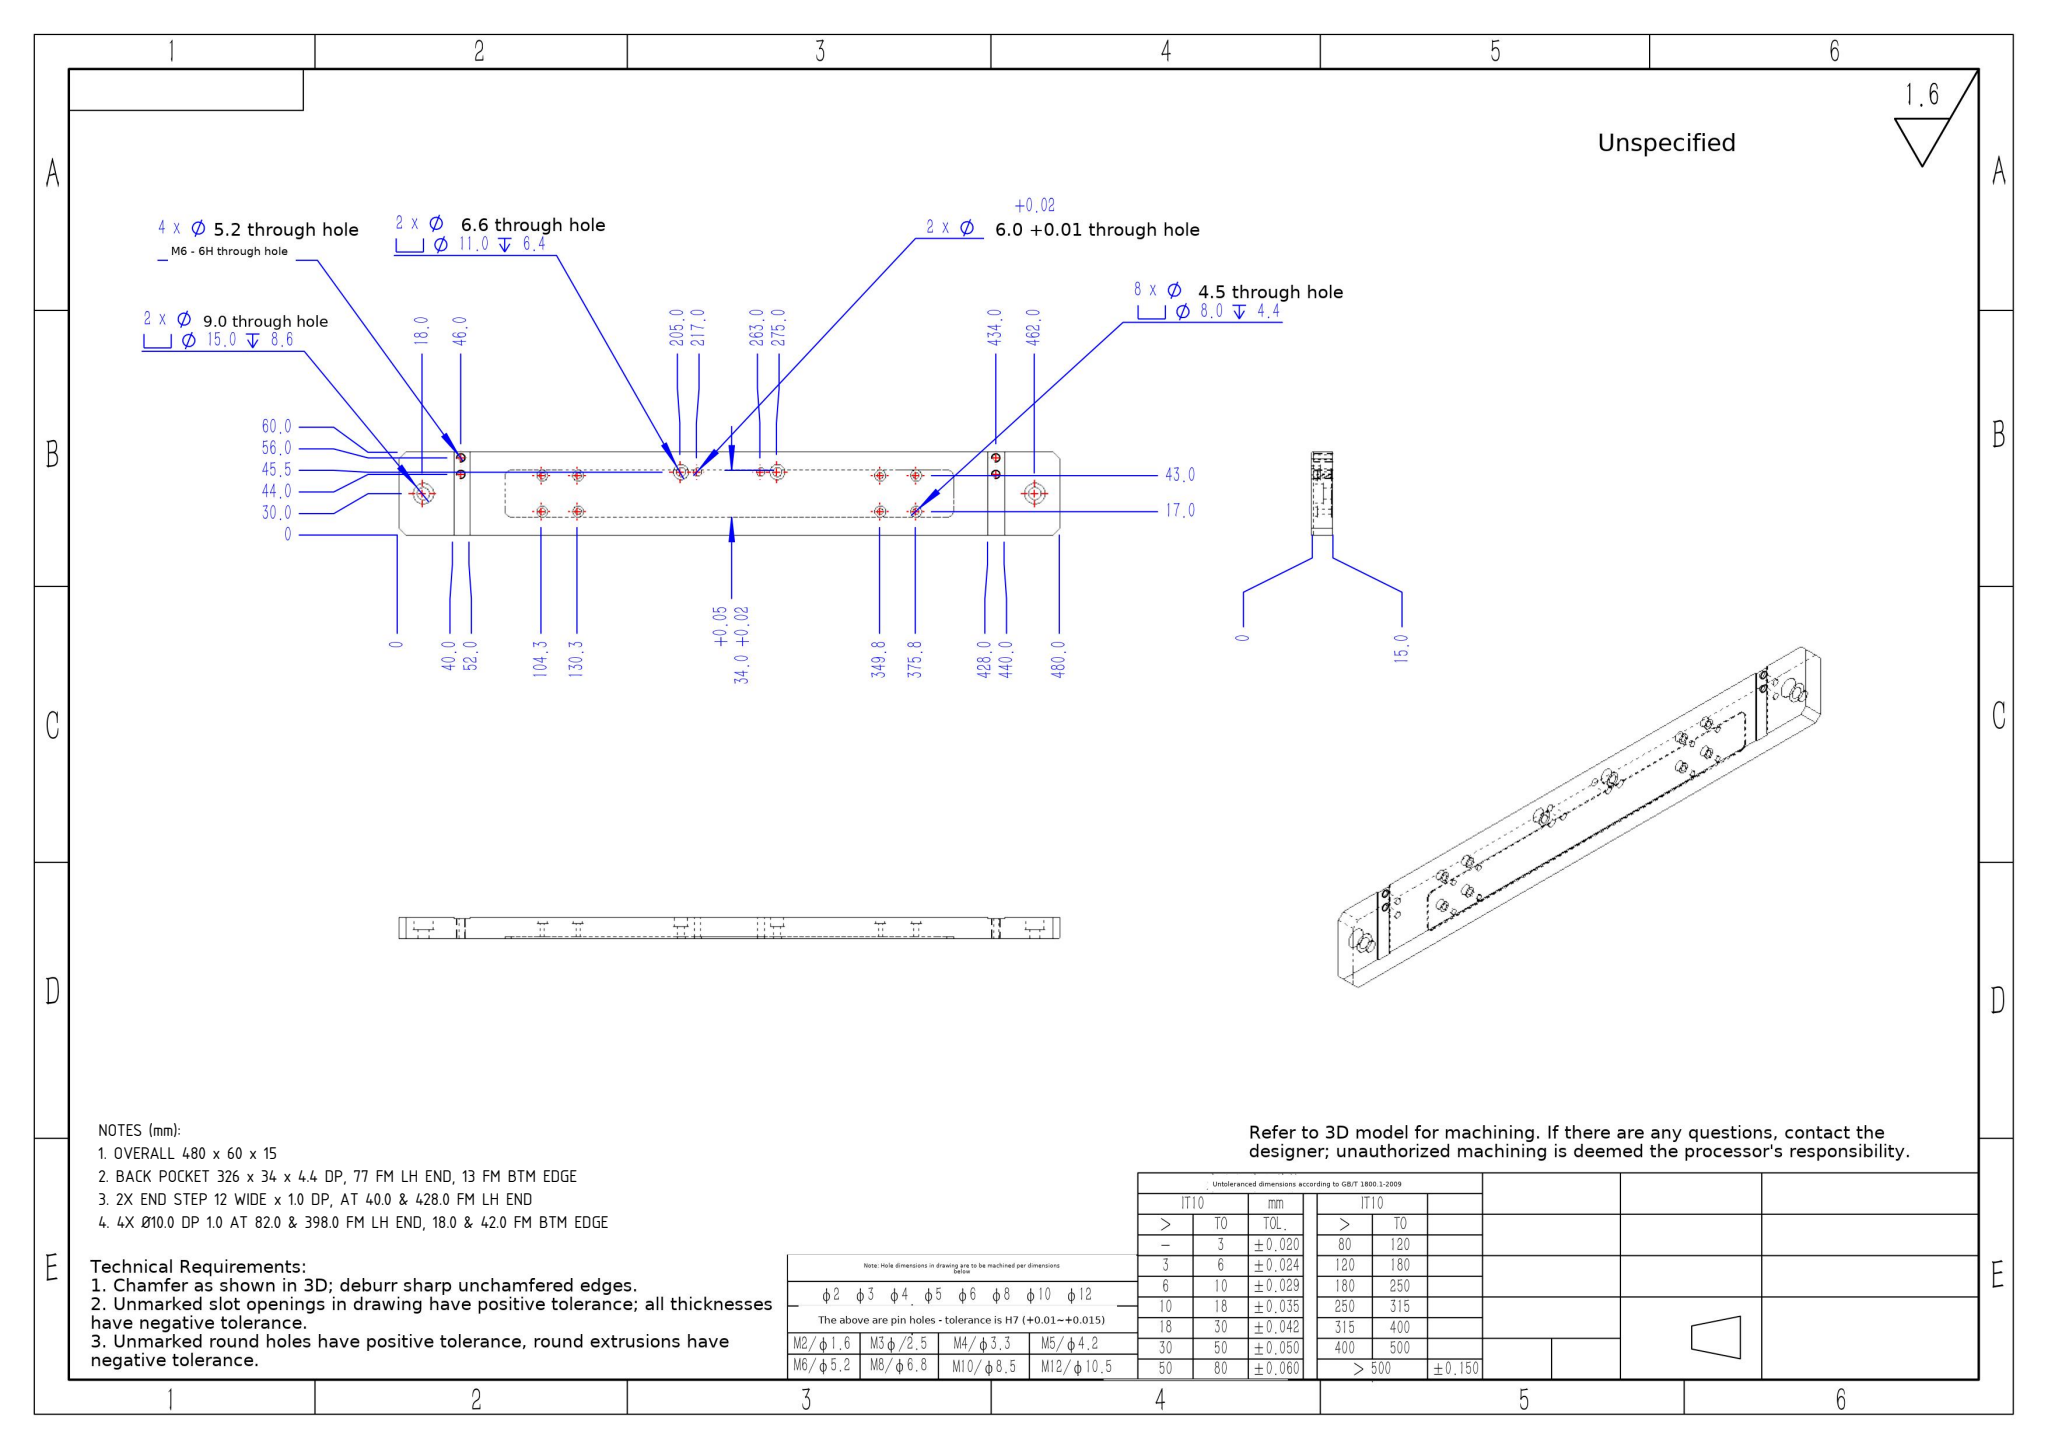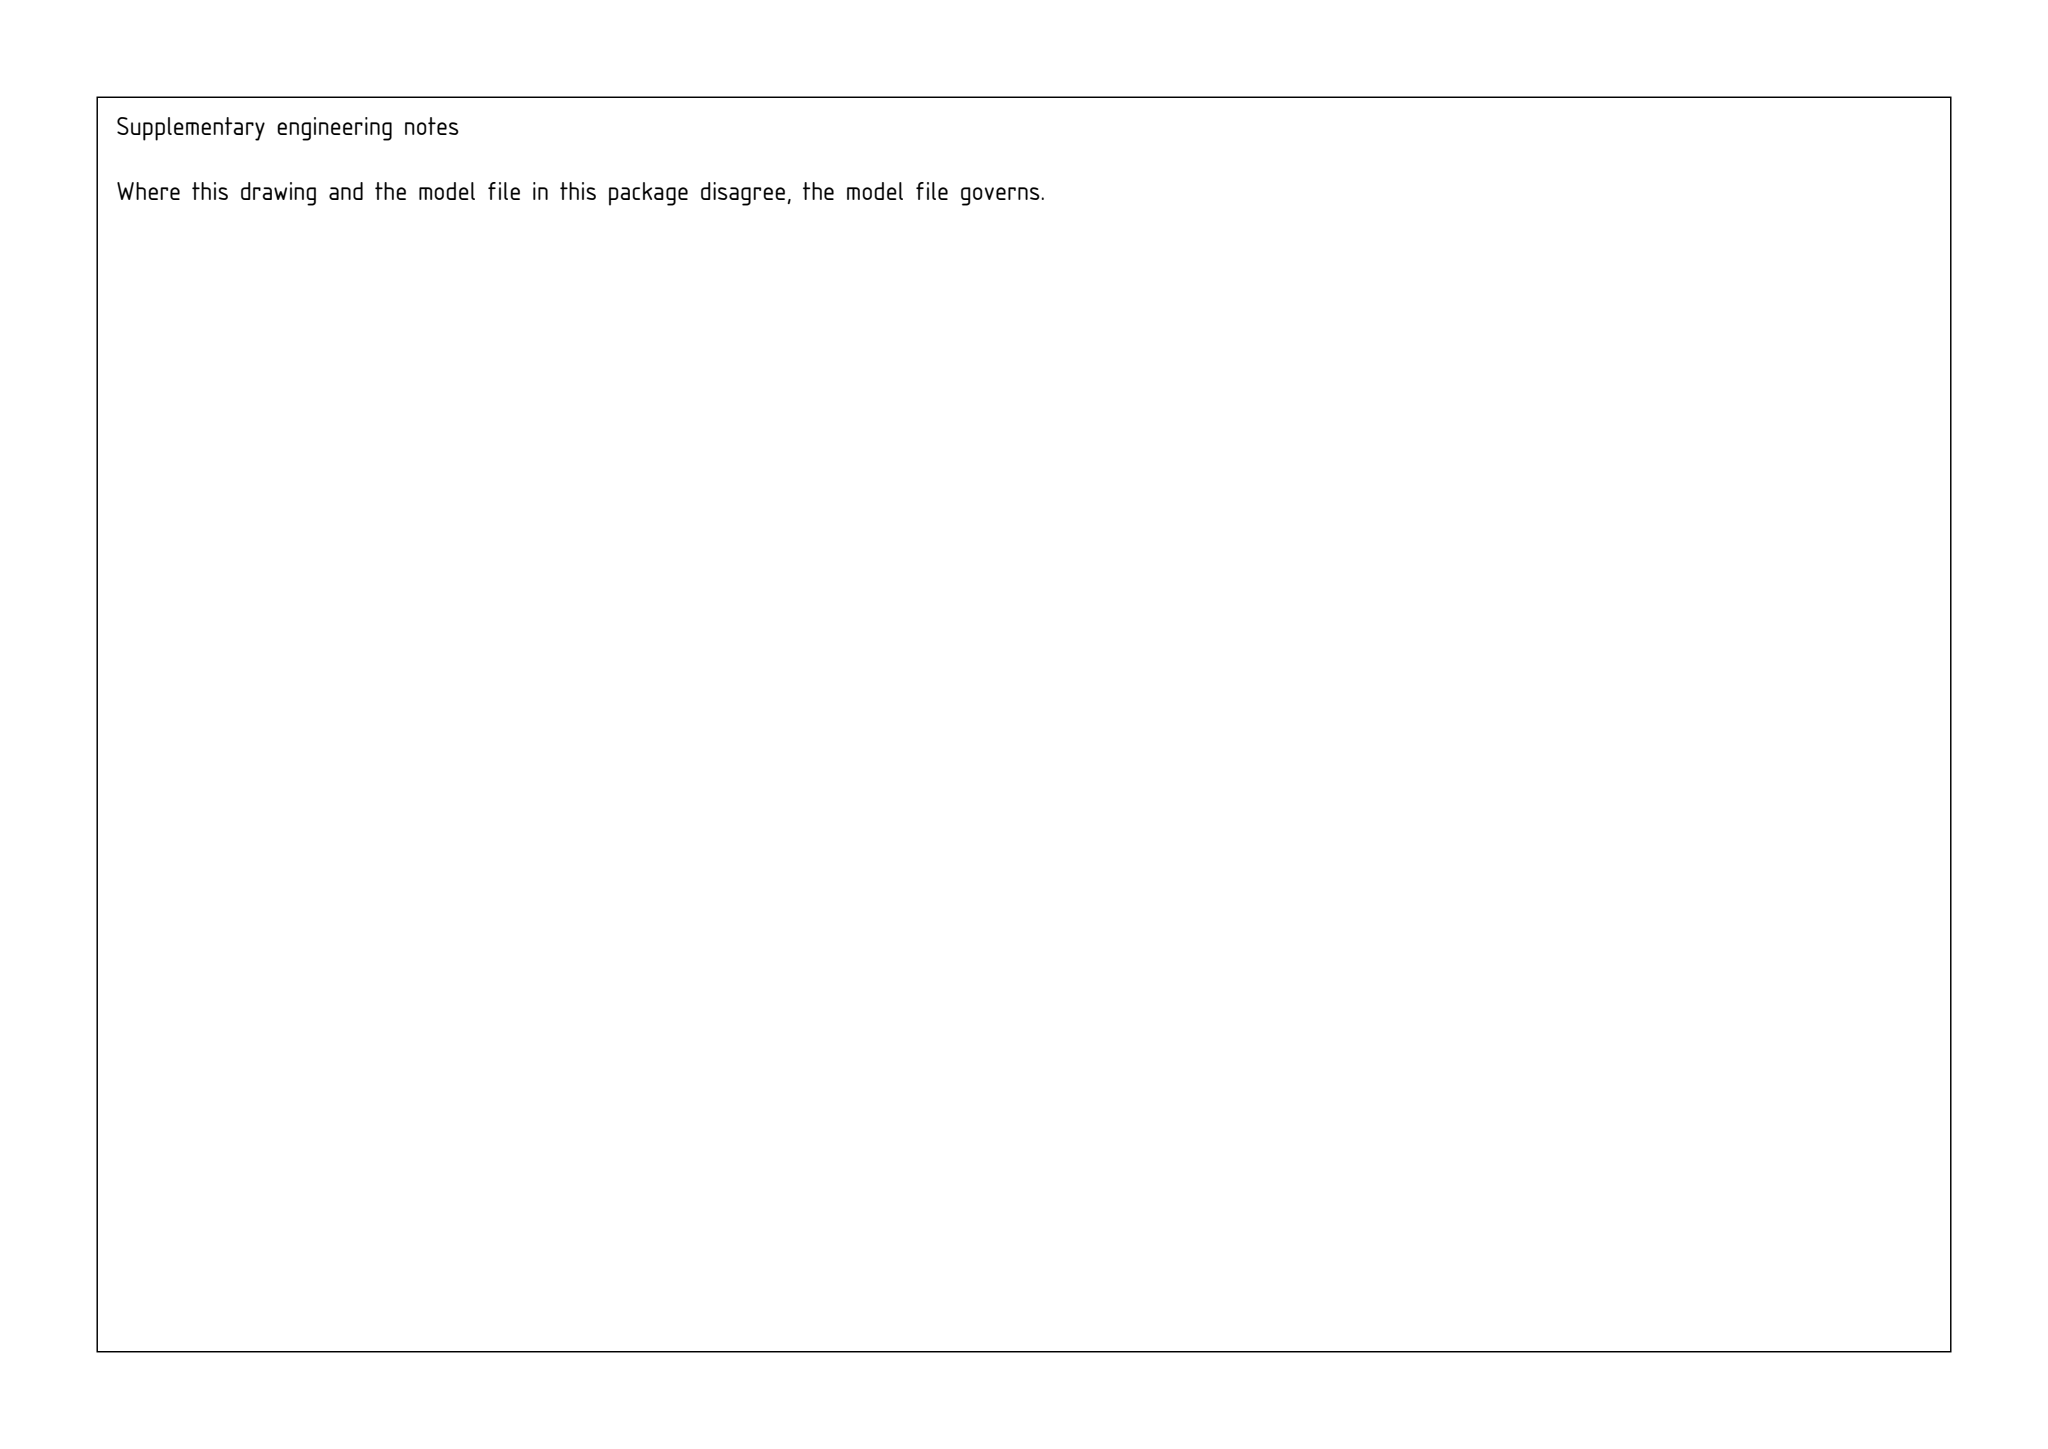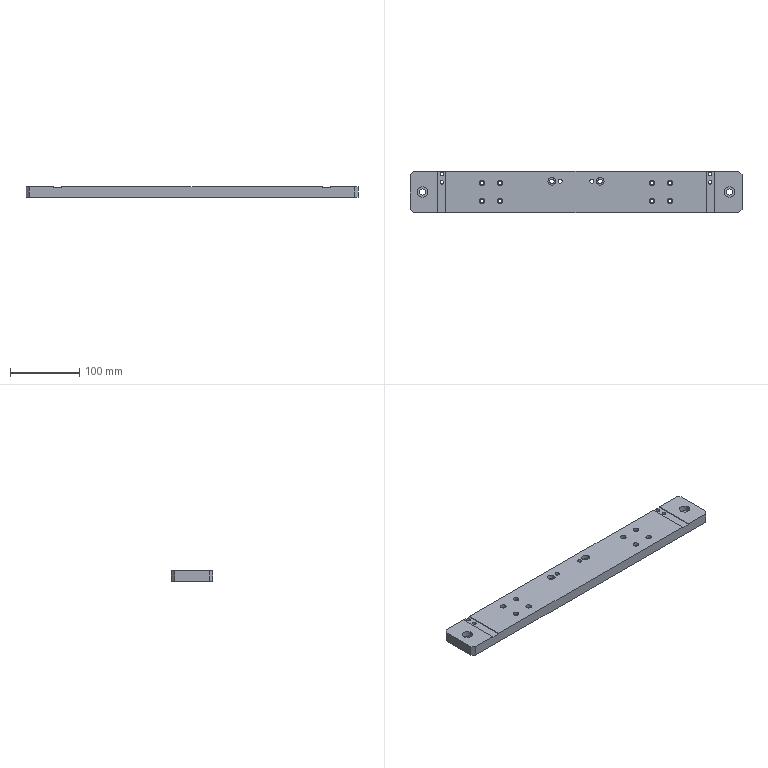Part | SolidWorks | mm | 1 solid | 103 faces | box 480 x 60 x 15 mm | volume 408159 mm3 | cylinder 64 | plane 39 | commonest cylinder face diameters 8 x16 4.5 x16 5.2 x8 6 x4 11 x4 6.6 x4 15 x4 9 x4
Drawing notes:
OVERALL 480 x 60 x 15 | from the solid: bbox_xyz 480.0 x 60.0 x 15.0
BACK POCKET 326 x 34 x 4.4 DP, 77 FM LH END, 13 FM BTM EDGE | from the solid: Planes x=77 & x=403 (326 lg), y=13 & y=47 (34 wide), floor z=10.6 vs face z=15.0
2X END STEP 12 WIDE x 1.0 DP, AT 40.0 & 428.0 FM LH END | from the solid: Planes x=40/52 & x=428/440; z=14.0 faces vs z=15.0 top (1.0 step)
4X Ø10.0 DP 1.0 AT 82.0 & 398.0 FM LH END, 18.0 & 42.0 FM BTM EDGE | from the solid: Ø10.0 z-cyls at [82,18],[82,42],[398,18],[398,42], len 1.0; z-plane 1.0
build123d program:
from build123d import *

# Parameters (mm, degrees)
SKETCH1_W                                       = 480
SKETCH1_H                                       = 60
BOSS_EXTRUDE1_DEPTH                             = 7.5
CHAMFER1_SIZE                                   = 5
SKETCH2_W                                       = 12
SKETCH2_H                                       = 60
CUT_EXTRUDE1_DEPTH                              = 1
M6_TAPPED_HOLE1_D                               = 5.2
M8_HEX_SOCKET_HEAD_CAP_SCREW_CBORE1_D           = 9
M8_HEX_SOCKET_HEAD_CAP_SCREW_CBORE1_CBORE_D     = 15
M8_HEX_SOCKET_HEAD_CAP_SCREW_CBORE1_CBORE_DEPTH = 8.6
SKETCH7_W                                       = 326
SKETCH7_H                                       = 34
CUT_EXTRUDE2_DEPTH                              = 1
FILLET1_R                                       = 5
M4_HEX_SOCKET_HEAD_CAP_SCREW_CBORE1_D           = 4.5
M4_HEX_SOCKET_HEAD_CAP_SCREW_CBORE1_DEPTH       = 15
M4_HEX_SOCKET_HEAD_CAP_SCREW_CBORE1_CBORE_D     = 8
M4_HEX_SOCKET_HEAD_CAP_SCREW_CBORE1_CBORE_DEPTH = 4.4
M6_HEX_SOCKET_HEAD_CAP_SCREW_CBORE1_D           = 6.6
M6_HEX_SOCKET_HEAD_CAP_SCREW_CBORE1_DEPTH       = 15
M6_HEX_SOCKET_HEAD_CAP_SCREW_CBORE1_CBORE_D     = 11
M6_HEX_SOCKET_HEAD_CAP_SCREW_CBORE1_CBORE_DEPTH = 6.4
SIZE_MM_DOWEL_HOLE1_D                           = 6
SIZE_MM_DOWEL_HOLE1_DEPTH                       = 15


with BuildPart() as part:
    # Sketch1 → Boss-Extrude1 (new, symmetric)
    with BuildSketch(Plane.XY):
        Rectangle(SKETCH1_W, SKETCH1_H)
    extrude(amount=BOSS_EXTRUDE1_DEPTH, both=True)

    # Chamfer1
    chamfer1_edges = [part.edges().sort_by_distance(p)[0] for p in [
        (240, -30, 0),
        (-240, -30, 0),
        (-240, 30, 0),
        (240, 30, 0),
    ]]
    chamfer(chamfer1_edges, length=CHAMFER1_SIZE)

    # Sketch2 → Cut-Extrude1 (cut)
    with BuildSketch(Plane.XY.offset(7.5)):
        with Locations((194, 0)):
            Rectangle(SKETCH2_W, SKETCH2_H)
    cut_extrude1 = extrude(amount=-CUT_EXTRUDE1_DEPTH, mode=Mode.SUBTRACT)

    # Mirror1: Cut-Extrude1 across plane
    add(cut_extrude1.mirror(Plane(origin=(0, 0, 0), x_dir=(0, 0, 1), z_dir=(1, 0, 0))), mode=Mode.SUBTRACT)

    # M6 Tapped Hole1 (through all)
    with Locations(Plane.XY.offset(7.5)):
        with Locations((-194, 14), (-194, 26), (194, 26), (194, 14)):
            Hole(M6_TAPPED_HOLE1_D / 2)

    # M8 Hex Socket Head Cap Screw CBORE1 (through all)
    with Locations(Plane.XY.offset(7.5)):
        with Locations((222, 0)):
            m8_hex_socket_head_cap_screw_cbore1 = CounterBoreHole(M8_HEX_SOCKET_HEAD_CAP_SCREW_CBORE1_D / 2, M8_HEX_SOCKET_HEAD_CAP_SCREW_CBORE1_CBORE_D / 2, M8_HEX_SOCKET_HEAD_CAP_SCREW_CBORE1_CBORE_DEPTH)

    # Mirror2: M8 Hex Socket Head Cap Screw CBORE1 across plane
    add(m8_hex_socket_head_cap_screw_cbore1.mirror(Plane(origin=(0, 0, 0), x_dir=(0, 0, 1), z_dir=(1, 0, 0))), mode=Mode.SUBTRACT)

    # Sketch7 → Cut-Extrude2 (cut)
    with BuildSketch(Plane(origin=(0, 0, -7.5), x_dir=(-1, 0, 0), z_dir=(0, 0, -1))):
        Rectangle(SKETCH7_W, SKETCH7_H)
    extrude(amount=-CUT_EXTRUDE2_DEPTH, mode=Mode.SUBTRACT)

    # Fillet1
    fillet1_edges = [part.edges().sort_by_distance(p)[0] for p in [
        (-163, 17, -7),
        (-163, -17, -7),
        (163, -17, -7),
        (163, 17, -7),
    ]]
    fillet(fillet1_edges, radius=FILLET1_R)

    # M4 Hex Socket Head Cap Screw CBORE1
    with Locations(Plane.XY.offset(7.5)):
        with Locations((-135.75, 13), (-109.75, 13), (-135.75, -13), (-109.75, -13), (109.75, 13), (135.75, 13), (109.75, -13), (135.75, -13)):
            CounterBoreHole(M4_HEX_SOCKET_HEAD_CAP_SCREW_CBORE1_D / 2, M4_HEX_SOCKET_HEAD_CAP_SCREW_CBORE1_CBORE_D / 2, M4_HEX_SOCKET_HEAD_CAP_SCREW_CBORE1_CBORE_DEPTH, depth=M4_HEX_SOCKET_HEAD_CAP_SCREW_CBORE1_DEPTH)

    # M6 Hex Socket Head Cap Screw CBORE1
    with Locations(Plane.XY.offset(7.5)):
        with Locations((35, 15.5), (-35, 15.5)):
            CounterBoreHole(M6_HEX_SOCKET_HEAD_CAP_SCREW_CBORE1_D / 2, M6_HEX_SOCKET_HEAD_CAP_SCREW_CBORE1_CBORE_D / 2, M6_HEX_SOCKET_HEAD_CAP_SCREW_CBORE1_CBORE_DEPTH, depth=M6_HEX_SOCKET_HEAD_CAP_SCREW_CBORE1_DEPTH)

    # Size mm Dowel Hole1
    with Locations(Plane.XY.offset(7.5)):
        with Locations((23, 15.5), (-23, 15.5)):
            Hole(SIZE_MM_DOWEL_HOLE1_D / 2, depth=SIZE_MM_DOWEL_HOLE1_DEPTH)


solid = part.part